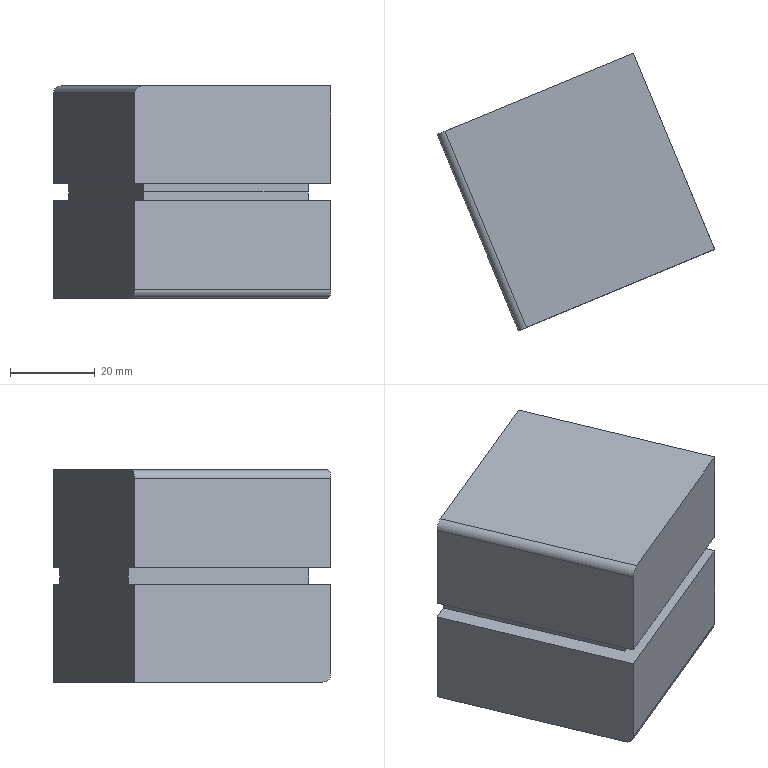Component | SolidWorks | Battery-2 | 1 solid | 17 faces | box 65.34 x 65.34 x 50 mm | volume 122620 mm3 | plane 15 | cylinder 2 | commonest cylinder face diameters 4 x2
build123d program:
from build123d import *

# Parameters (mm, degrees)
SKETCH1_W           = 50
SKETCH1_H           = 50
BOSS_EXTRUDE1_DEPTH = 50
SKETCH8_W           = 4
SKETCH8_H           = 4
FILLET1_R           = 2
FILLET4_R           = 2


with BuildPart() as part:
    # Sketch1 → Boss-Extrude1 (new body)
    with BuildSketch(Plane(origin=(0, 0, 0), x_dir=(1, 0, 0), z_dir=(0, 1, 0))):
        with Locations((0.8865, -4.255)):
            Rectangle(SKETCH1_W, SKETCH1_H)
    extrude(amount=BOSS_EXTRUDE1_DEPTH)

    # Cut-Sweep2: sweep along a path in Sketch2
    with BuildLine(Plane(origin=(25.887, 0, 0), x_dir=(0, 0, -1), z_dir=(1, 0, 0))) as cut_sweep2_path:
        Line((-4.255, 50), (-4.255, 0))
    # Sketch7 → Cut-Sweep2 (sweep, cut)
    with BuildSketch(Plane.XZ):
        Polygon((25.887, 4.255), (25.887, 6.255), (21.763, 6.255), (21.763, 2.255), (25.887, 2.255), align=None)
    sweep(path=cut_sweep2_path.line, mode=Mode.SUBTRACT)

    # Cut-Sweep3: sweep along a path in Sketch4
    with BuildLine(Plane.ZY.offset(24.113)) as cut_sweep3_path:
        Line((4.255, 50), (4.255, 0))
    # Sketch8 → Cut-Sweep3 (sweep, cut)
    with BuildSketch(Plane.XZ):
        with Locations((-22.117, 4.255)):
            Rectangle(SKETCH8_W, SKETCH8_H)
    sweep(path=cut_sweep3_path.line, mode=Mode.SUBTRACT)

    # Cut-Sweep4: sweep along a path in Sketch5
    with BuildLine(Plane.XZ) as cut_sweep4_path:
        Line((25.887, 4.255), (-24.113, 4.255))
    # Sketch10 → Cut-Sweep4 (sweep, cut)
    with BuildSketch(Plane(origin=(25.887, 0, 0), x_dir=(0, 0, -1), z_dir=(1, 0, 0))):
        Polygon((-2.255, 0), (-2.255, 4), (-4.255, 4), (-6.255, 4), (-6.255, 0), align=None)
    sweep(path=cut_sweep4_path.line, mode=Mode.SUBTRACT)

    # Fillet1
    fillet1_edges = [part.edges().sort_by_distance(p)[0] for p in [
        (-24.113, 25, 29.255),
    ]]
    fillet(fillet1_edges, radius=FILLET1_R)

    # Fillet4
    fillet4_edges = [part.edges().sort_by_distance(p)[0] for p in [
        (0.8865, 0, -20.745),
    ]]
    fillet(fillet4_edges, radius=FILLET4_R)


solid = part.part

# Placed as in the assembly
solid = solid.moved(Location((39.632, -16.373, 266.591), (0, 0, 22.523)))
STEP:
#1=COLOUR_RGB('',0.7922,0.8196,0.9333);
#2=FILL_AREA_STYLE_COLOUR('',#1);
#3=FILL_AREA_STYLE('',(#2));
#4=SURFACE_STYLE_FILL_AREA(#3);
#5=SURFACE_SIDE_STYLE('',(#4));
#6=SURFACE_STYLE_USAGE(.BOTH.,#5);
#7=PRESENTATION_STYLE_ASSIGNMENT((#6));
#8=CARTESIAN_POINT('',(0.7561,-0.9781,11.647));
#9=VERTEX_POINT('',#8);
#10=CARTESIAN_POINT('',(2.502,-0.2542,11.647));
#11=VERTEX_POINT('',#10);
#12=CARTESIAN_POINT('',(0.6834,-1.008,11.647));
#13=DIRECTION('',(0.9237,0.383,0.));
#14=VECTOR('',#13,39.37);
#15=LINE('',#12,#14);
#16=EDGE_CURVE('',#9,#11,#15,.T.);
#17=ORIENTED_EDGE('',*,*,#16,.F.);
#18=CARTESIAN_POINT('',(0.6834,-1.008,11.569));
#19=VERTEX_POINT('',#18);
#20=CARTESIAN_POINT('',(0.7561,-0.9781,11.569));
#21=DIRECTION('',(0.383,-0.9237,0.));
#22=DIRECTION('',(0.,0.,1.));
#23=AXIS2_PLACEMENT_3D('',#20,#21,#22);
#24=CIRCLE('',#23,0.07874);
#25=EDGE_CURVE('',#9,#19,#24,.T.);
#26=ORIENTED_EDGE('',*,*,#25,.T.);
#27=CARTESIAN_POINT('',(0.6834,-1.008,10.742));
#28=VERTEX_POINT('',#27);
#29=CARTESIAN_POINT('',(0.6834,-1.008,9.679));
#30=DIRECTION('',(-0.,-0.,1.));
#31=VECTOR('',#30,39.37);
#32=LINE('',#29,#31);
#33=EDGE_CURVE('',#28,#19,#32,.T.);
#34=ORIENTED_EDGE('',*,*,#33,.F.);
#35=CARTESIAN_POINT('',(2.502,-0.2542,10.742));
#36=VERTEX_POINT('',#35);
#37=CARTESIAN_POINT('',(2.502,-0.2542,10.742));
#38=DIRECTION('',(-0.9237,-0.383,-0.));
#39=VECTOR('',#38,39.37);
#40=LINE('',#37,#39);
#41=EDGE_CURVE('',#36,#28,#40,.T.);
#42=ORIENTED_EDGE('',*,*,#41,.F.);
#43=CARTESIAN_POINT('',(2.502,-0.2542,9.679));
#44=DIRECTION('',(0.,0.,-1.));
#45=VECTOR('',#44,39.37);
#46=LINE('',#43,#45);
#47=EDGE_CURVE('',#11,#36,#46,.T.);
#48=ORIENTED_EDGE('',*,*,#47,.F.);
#49=EDGE_LOOP('',(#17,#26,#34,#42,#48));
#50=FACE_OUTER_BOUND('',#49,.T.);
#51=CARTESIAN_POINT('',(1.56,-0.6446,10.496));
#52=DIRECTION('',(-0.383,0.9237,-0.));
#53=DIRECTION('',(-0.,-0.,1.));
#54=AXIS2_PLACEMENT_3D('',#51,#52,#53);
#55=PLANE('',#54);
#56=ADVANCED_FACE('',(#50),#55,.F.);
#57=CARTESIAN_POINT('',(2.291,-0.1709,10.584));
#58=VERTEX_POINT('',#57);
#59=CARTESIAN_POINT('',(2.291,-0.1709,10.663));
#60=VERTEX_POINT('',#59);
#61=CARTESIAN_POINT('',(2.291,-0.1709,10.742));
#62=DIRECTION('',(-0.,-0.,1.));
#63=VECTOR('',#62,39.37);
#64=LINE('',#61,#63);
#65=EDGE_CURVE('',#58,#60,#64,.T.);
#66=ORIENTED_EDGE('',*,*,#65,.F.);
#67=CARTESIAN_POINT('',(1.598,1.502,10.584));
#68=VERTEX_POINT('',#67);
#69=CARTESIAN_POINT('',(1.583,1.538,10.584));
#70=DIRECTION('',(0.383,-0.9237,-0.));
#71=VECTOR('',#70,39.37);
#72=LINE('',#69,#71);
#73=EDGE_CURVE('',#68,#58,#72,.T.);
#74=ORIENTED_EDGE('',*,*,#73,.F.);
#75=CARTESIAN_POINT('',(1.598,1.502,10.742));
#76=VERTEX_POINT('',#75);
#77=CARTESIAN_POINT('',(1.598,1.502,10.742));
#78=DIRECTION('',(0.,0.,-1.));
#79=VECTOR('',#78,39.37);
#80=LINE('',#77,#79);
#81=EDGE_CURVE('',#76,#68,#80,.T.);
#82=ORIENTED_EDGE('',*,*,#81,.F.);
#83=CARTESIAN_POINT('',(2.291,-0.1709,10.742));
#84=VERTEX_POINT('',#83);
#85=CARTESIAN_POINT('',(1.583,1.538,10.742));
#86=DIRECTION('',(0.383,-0.9237,-0.));
#87=VECTOR('',#86,39.37);
#88=LINE('',#85,#87);
#89=EDGE_CURVE('',#76,#84,#88,.T.);
#90=ORIENTED_EDGE('',*,*,#89,.T.);
#91=CARTESIAN_POINT('',(2.291,-0.1709,10.742));
#92=DIRECTION('',(-0.,-0.,1.));
#93=VECTOR('',#92,39.37);
#94=LINE('',#91,#93);
#95=EDGE_CURVE('',#60,#84,#94,.T.);
#96=ORIENTED_EDGE('',*,*,#95,.F.);
#97=EDGE_LOOP('',(#66,#74,#82,#90,#96));
#98=FACE_OUTER_BOUND('',#97,.T.);
#99=CARTESIAN_POINT('',(1.583,1.538,10.742));
#100=DIRECTION('',(-0.9237,-0.383,-0.));
#101=DIRECTION('',(-0.,-0.,1.));
#102=AXIS2_PLACEMENT_3D('',#99,#100,#101);
#103=PLANE('',#102);
#104=ADVANCED_FACE('',(#98),#103,.F.);
#105=CARTESIAN_POINT('',(0.7684,-0.8025,10.663));
#106=VERTEX_POINT('',#105);
#107=CARTESIAN_POINT('',(0.7684,-0.8025,10.584));
#108=VERTEX_POINT('',#107);
#109=CARTESIAN_POINT('',(0.7684,-0.8025,10.742));
#110=DIRECTION('',(0.,0.,-1.));
#111=VECTOR('',#110,39.37);
#112=LINE('',#109,#111);
#113=EDGE_CURVE('',#106,#108,#112,.T.);
#114=ORIENTED_EDGE('',*,*,#113,.F.);
#115=CARTESIAN_POINT('',(0.7684,-0.8025,10.742));
#116=VERTEX_POINT('',#115);
#117=CARTESIAN_POINT('',(0.7684,-0.8025,10.742));
#118=DIRECTION('',(0.,0.,-1.));
#119=VECTOR('',#118,39.37);
#120=LINE('',#117,#119);
#121=EDGE_CURVE('',#116,#106,#120,.T.);
#122=ORIENTED_EDGE('',*,*,#121,.F.);
#123=CARTESIAN_POINT('',(0.07469,0.8704,10.742));
#124=VERTEX_POINT('',#123);
#125=CARTESIAN_POINT('',(0.05961,0.9067,10.742));
#126=DIRECTION('',(0.383,-0.9237,-0.));
#127=VECTOR('',#126,39.37);
#128=LINE('',#125,#127);
#129=EDGE_CURVE('',#124,#116,#128,.T.);
#130=ORIENTED_EDGE('',*,*,#129,.F.);
#131=CARTESIAN_POINT('',(0.07469,0.8704,10.584));
#132=VERTEX_POINT('',#131);
#133=CARTESIAN_POINT('',(0.07469,0.8704,10.742));
#134=DIRECTION('',(-0.,-0.,1.));
#135=VECTOR('',#134,39.37);
#136=LINE('',#133,#135);
#137=EDGE_CURVE('',#132,#124,#136,.T.);
#138=ORIENTED_EDGE('',*,*,#137,.F.);
#139=CARTESIAN_POINT('',(0.05961,0.9067,10.584));
#140=DIRECTION('',(0.383,-0.9237,-0.));
#141=VECTOR('',#140,39.37);
#142=LINE('',#139,#141);
#143=EDGE_CURVE('',#132,#108,#142,.T.);
#144=ORIENTED_EDGE('',*,*,#143,.T.);
#145=EDGE_LOOP('',(#114,#122,#130,#138,#144));
#146=FACE_OUTER_BOUND('',#145,.T.);
#147=CARTESIAN_POINT('',(0.05961,0.9067,10.742));
#148=DIRECTION('',(0.9237,0.383,0.));
#149=DIRECTION('',(0.,0.,-1.));
#150=AXIS2_PLACEMENT_3D('',#147,#148,#149);
#151=PLANE('',#150);
#152=ADVANCED_FACE('',(#146),#151,.F.);
#153=ORIENTED_EDGE('',*,*,#33,.T.);
#154=CARTESIAN_POINT('',(-0.07064,0.8101,11.569));
#155=VERTEX_POINT('',#154);
#156=CARTESIAN_POINT('',(-0.07064,0.8101,11.569));
#157=DIRECTION('',(-0.383,0.9237,-0.));
#158=VECTOR('',#157,39.37);
#159=LINE('',#156,#158);
#160=EDGE_CURVE('',#19,#155,#159,.T.);
#161=ORIENTED_EDGE('',*,*,#160,.T.);
#162=CARTESIAN_POINT('',(-0.07064,0.8101,10.742));
#163=VERTEX_POINT('',#162);
#164=CARTESIAN_POINT('',(-0.07064,0.8101,9.679));
#165=DIRECTION('',(-0.,-0.,1.));
#166=VECTOR('',#165,39.37);
#167=LINE('',#164,#166);
#168=EDGE_CURVE('',#163,#155,#167,.T.);
#169=ORIENTED_EDGE('',*,*,#168,.F.);
#170=CARTESIAN_POINT('',(-0.07064,0.8101,10.742));
#171=DIRECTION('',(0.383,-0.9237,-0.));
#172=VECTOR('',#171,39.37);
#173=LINE('',#170,#172);
#174=EDGE_CURVE('',#163,#28,#173,.T.);
#175=ORIENTED_EDGE('',*,*,#174,.T.);
#176=EDGE_LOOP('',(#153,#161,#169,#175));
#177=FACE_OUTER_BOUND('',#176,.T.);
#178=CARTESIAN_POINT('',(-0.07064,0.8101,9.679));
#179=DIRECTION('',(0.9237,0.383,0.));
#180=DIRECTION('',(0.,0.,-1.));
#181=AXIS2_PLACEMENT_3D('',#178,#179,#180);
#182=PLANE('',#181);
#183=ADVANCED_FACE('',(#177),#182,.F.);
#184=CARTESIAN_POINT('',(2.502,-0.2542,10.584));
#185=VERTEX_POINT('',#184);
#186=CARTESIAN_POINT('',(2.502,-0.2542,9.758));
#187=VERTEX_POINT('',#186);
#188=CARTESIAN_POINT('',(2.502,-0.2542,9.679));
#189=DIRECTION('',(0.,0.,-1.));
#190=VECTOR('',#189,39.37);
#191=LINE('',#188,#190);
#192=EDGE_CURVE('',#185,#187,#191,.T.);
#193=ORIENTED_EDGE('',*,*,#192,.T.);
#194=CARTESIAN_POINT('',(2.472,-0.1815,9.679));
#195=VERTEX_POINT('',#194);
#196=CARTESIAN_POINT('',(2.472,-0.1815,9.758));
#197=DIRECTION('',(0.9237,0.383,0.));
#198=DIRECTION('',(0.,0.,1.));
#199=AXIS2_PLACEMENT_3D('',#196,#197,#198);
#200=CIRCLE('',#199,0.07874);
#201=EDGE_CURVE('',#187,#195,#200,.T.);
#202=ORIENTED_EDGE('',*,*,#201,.T.);
#203=CARTESIAN_POINT('',(1.748,1.564,9.679));
#204=VERTEX_POINT('',#203);
#205=CARTESIAN_POINT('',(1.748,1.564,9.679));
#206=DIRECTION('',(0.383,-0.9237,0.));
#207=VECTOR('',#206,39.37);
#208=LINE('',#205,#207);
#209=EDGE_CURVE('',#204,#195,#208,.T.);
#210=ORIENTED_EDGE('',*,*,#209,.F.);
#211=CARTESIAN_POINT('',(1.748,1.564,10.584));
#212=VERTEX_POINT('',#211);
#213=CARTESIAN_POINT('',(1.748,1.564,9.679));
#214=DIRECTION('',(0.,0.,-1.));
#215=VECTOR('',#214,39.37);
#216=LINE('',#213,#215);
#217=EDGE_CURVE('',#212,#204,#216,.T.);
#218=ORIENTED_EDGE('',*,*,#217,.F.);
#219=CARTESIAN_POINT('',(1.733,1.601,10.584));
#220=DIRECTION('',(0.383,-0.9237,-0.));
#221=VECTOR('',#220,39.37);
#222=LINE('',#219,#221);
#223=EDGE_CURVE('',#212,#185,#222,.T.);
#224=ORIENTED_EDGE('',*,*,#223,.T.);
#225=EDGE_LOOP('',(#193,#202,#210,#218,#224));
#226=FACE_OUTER_BOUND('',#225,.T.);
#227=CARTESIAN_POINT('',(1.748,1.564,9.679));
#228=DIRECTION('',(-0.9237,-0.383,-0.));
#229=DIRECTION('',(-0.,-0.,1.));
#230=AXIS2_PLACEMENT_3D('',#227,#228,#229);
#231=PLANE('',#230);
#232=ADVANCED_FACE('',(#226),#231,.F.);
#233=CARTESIAN_POINT('',(-0.07064,0.8101,9.679));
#234=VERTEX_POINT('',#233);
#235=CARTESIAN_POINT('',(0.6532,-0.9355,9.679));
#236=VERTEX_POINT('',#235);
#237=CARTESIAN_POINT('',(-0.07064,0.8101,9.679));
#238=DIRECTION('',(0.383,-0.9237,0.));
#239=VECTOR('',#238,39.37);
#240=LINE('',#237,#239);
#241=EDGE_CURVE('',#234,#236,#240,.T.);
#242=ORIENTED_EDGE('',*,*,#241,.T.);
#243=CARTESIAN_POINT('',(0.6834,-1.008,9.758));
#244=VERTEX_POINT('',#243);
#245=CARTESIAN_POINT('',(0.6532,-0.9355,9.758));
#246=DIRECTION('',(-0.9237,-0.383,-0.));
#247=DIRECTION('',(0.,0.,-1.));
#248=AXIS2_PLACEMENT_3D('',#245,#246,#247);
#249=CIRCLE('',#248,0.07874);
#250=EDGE_CURVE('',#236,#244,#249,.T.);
#251=ORIENTED_EDGE('',*,*,#250,.T.);
#252=CARTESIAN_POINT('',(0.6834,-1.008,10.584));
#253=VERTEX_POINT('',#252);
#254=CARTESIAN_POINT('',(0.6834,-1.008,9.679));
#255=DIRECTION('',(-0.,-0.,1.));
#256=VECTOR('',#255,39.37);
#257=LINE('',#254,#256);
#258=EDGE_CURVE('',#244,#253,#257,.T.);
#259=ORIENTED_EDGE('',*,*,#258,.T.);
#260=CARTESIAN_POINT('',(-0.07064,0.8101,10.584));
#261=VERTEX_POINT('',#260);
#262=CARTESIAN_POINT('',(-0.07064,0.8101,10.584));
#263=DIRECTION('',(-0.383,0.9237,0.));
#264=VECTOR('',#263,39.37);
#265=LINE('',#262,#264);
#266=EDGE_CURVE('',#253,#261,#265,.T.);
#267=ORIENTED_EDGE('',*,*,#266,.T.);
#268=CARTESIAN_POINT('',(-0.07064,0.8101,9.679));
#269=DIRECTION('',(-0.,-0.,1.));
#270=VECTOR('',#269,39.37);
#271=LINE('',#268,#270);
#272=EDGE_CURVE('',#234,#261,#271,.T.);
#273=ORIENTED_EDGE('',*,*,#272,.F.);
#274=EDGE_LOOP('',(#242,#251,#259,#267,#273));
#275=FACE_OUTER_BOUND('',#274,.T.);
#276=CARTESIAN_POINT('',(-0.07064,0.8101,9.679));
#277=DIRECTION('',(0.9237,0.383,0.));
#278=DIRECTION('',(0.,0.,-1.));
#279=AXIS2_PLACEMENT_3D('',#276,#277,#278);
#280=PLANE('',#279);
#281=ADVANCED_FACE('',(#275),#280,.F.);
#282=CARTESIAN_POINT('',(0.002094,0.8403,11.647));
#283=VERTEX_POINT('',#282);
#284=CARTESIAN_POINT('',(1.748,1.564,11.647));
#285=VERTEX_POINT('',#284);
#286=CARTESIAN_POINT('',(-0.07064,0.8101,11.647));
#287=DIRECTION('',(0.9237,0.383,0.));
#288=VECTOR('',#287,39.37);
#289=LINE('',#286,#288);
#290=EDGE_CURVE('',#283,#285,#289,.T.);
#291=ORIENTED_EDGE('',*,*,#290,.F.);
#292=CARTESIAN_POINT('',(0.002094,0.8403,11.647));
#293=DIRECTION('',(0.383,-0.9237,0.));
#294=VECTOR('',#293,39.37);
#295=LINE('',#292,#294);
#296=EDGE_CURVE('',#283,#9,#295,.T.);
#297=ORIENTED_EDGE('',*,*,#296,.T.);
#298=ORIENTED_EDGE('',*,*,#16,.T.);
#299=CARTESIAN_POINT('',(1.748,1.564,11.647));
#300=DIRECTION('',(0.383,-0.9237,0.));
#301=VECTOR('',#300,39.37);
#302=LINE('',#299,#301);
#303=EDGE_CURVE('',#285,#11,#302,.T.);
#304=ORIENTED_EDGE('',*,*,#303,.F.);
#305=EDGE_LOOP('',(#291,#297,#298,#304));
#306=FACE_OUTER_BOUND('',#305,.T.);
#307=CARTESIAN_POINT('',(-0.07064,0.8101,11.647));
#308=DIRECTION('',(0.,0.,-1.));
#309=DIRECTION('',(-0.9237,-0.383,-0.));
#310=AXIS2_PLACEMENT_3D('',#307,#308,#309);
#311=PLANE('',#310);
#312=ADVANCED_FACE('',(#306),#311,.F.);
#313=ORIENTED_EDGE('',*,*,#47,.T.);
#314=CARTESIAN_POINT('',(1.748,1.564,10.742));
#315=VERTEX_POINT('',#314);
#316=CARTESIAN_POINT('',(1.733,1.601,10.742));
#317=DIRECTION('',(0.383,-0.9237,-0.));
#318=VECTOR('',#317,39.37);
#319=LINE('',#316,#318);
#320=EDGE_CURVE('',#315,#36,#319,.T.);
#321=ORIENTED_EDGE('',*,*,#320,.F.);
#322=CARTESIAN_POINT('',(1.748,1.564,9.679));
#323=DIRECTION('',(0.,0.,-1.));
#324=VECTOR('',#323,39.37);
#325=LINE('',#322,#324);
#326=EDGE_CURVE('',#285,#315,#325,.T.);
#327=ORIENTED_EDGE('',*,*,#326,.F.);
#328=ORIENTED_EDGE('',*,*,#303,.T.);
#329=EDGE_LOOP('',(#313,#321,#327,#328));
#330=FACE_OUTER_BOUND('',#329,.T.);
#331=CARTESIAN_POINT('',(1.748,1.564,9.679));
#332=DIRECTION('',(-0.9237,-0.383,-0.));
#333=DIRECTION('',(-0.,-0.,1.));
#334=AXIS2_PLACEMENT_3D('',#331,#332,#333);
#335=PLANE('',#334);
#336=ADVANCED_FACE('',(#330),#335,.F.);
#337=ORIENTED_EDGE('',*,*,#209,.T.);
#338=CARTESIAN_POINT('',(0.6532,-0.9355,9.679));
#339=DIRECTION('',(-0.9237,-0.383,-0.));
#340=VECTOR('',#339,39.37);
#341=LINE('',#338,#340);
#342=EDGE_CURVE('',#195,#236,#341,.T.);
#343=ORIENTED_EDGE('',*,*,#342,.T.);
#344=ORIENTED_EDGE('',*,*,#241,.F.);
#345=CARTESIAN_POINT('',(-0.07064,0.8101,9.679));
#346=DIRECTION('',(-0.9237,-0.383,-0.));
#347=VECTOR('',#346,39.37);
#348=LINE('',#345,#347);
#349=EDGE_CURVE('',#204,#234,#348,.T.);
#350=ORIENTED_EDGE('',*,*,#349,.F.);
#351=EDGE_LOOP('',(#337,#343,#344,#350));
#352=FACE_OUTER_BOUND('',#351,.T.);
#353=CARTESIAN_POINT('',(-0.07064,0.8101,9.679));
#354=DIRECTION('',(-0.,-0.,1.));
#355=DIRECTION('',(0.9237,0.383,0.));
#356=AXIS2_PLACEMENT_3D('',#353,#354,#355);
#357=PLANE('',#356);
#358=ADVANCED_FACE('',(#352),#357,.F.);
#359=ORIENTED_EDGE('',*,*,#168,.T.);
#360=CARTESIAN_POINT('',(0.002094,0.8403,11.569));
#361=DIRECTION('',(-0.383,0.9237,-0.));
#362=DIRECTION('',(-0.,0.,1.));
#363=AXIS2_PLACEMENT_3D('',#360,#361,#362);
#364=CIRCLE('',#363,0.07874);
#365=EDGE_CURVE('',#155,#283,#364,.T.);
#366=ORIENTED_EDGE('',*,*,#365,.T.);
#367=ORIENTED_EDGE('',*,*,#290,.T.);
#368=ORIENTED_EDGE('',*,*,#326,.T.);
#369=CARTESIAN_POINT('',(1.748,1.564,10.742));
#370=DIRECTION('',(-0.9237,-0.383,-0.));
#371=VECTOR('',#370,39.37);
#372=LINE('',#369,#371);
#373=EDGE_CURVE('',#315,#76,#372,.T.);
#374=ORIENTED_EDGE('',*,*,#373,.T.);
#375=ORIENTED_EDGE('',*,*,#81,.T.);
#376=CARTESIAN_POINT('',(1.598,1.502,10.584));
#377=DIRECTION('',(0.9237,0.383,0.));
#378=VECTOR('',#377,39.37);
#379=LINE('',#376,#378);
#380=EDGE_CURVE('',#68,#212,#379,.T.);
#381=ORIENTED_EDGE('',*,*,#380,.T.);
#382=ORIENTED_EDGE('',*,*,#217,.T.);
#383=ORIENTED_EDGE('',*,*,#349,.T.);
#384=ORIENTED_EDGE('',*,*,#272,.T.);
#385=CARTESIAN_POINT('',(-0.07078,0.8101,10.584));
#386=DIRECTION('',(0.9237,0.383,0.));
#387=VECTOR('',#386,39.37);
#388=LINE('',#385,#387);
#389=EDGE_CURVE('',#261,#132,#388,.T.);
#390=ORIENTED_EDGE('',*,*,#389,.T.);
#391=ORIENTED_EDGE('',*,*,#137,.T.);
#392=CARTESIAN_POINT('',(0.07469,0.8704,10.742));
#393=DIRECTION('',(-0.9237,-0.383,-0.));
#394=VECTOR('',#393,39.37);
#395=LINE('',#392,#394);
#396=EDGE_CURVE('',#124,#163,#395,.T.);
#397=ORIENTED_EDGE('',*,*,#396,.T.);
#398=EDGE_LOOP('',(#359,#366,#367,#368,#374,#375,#381,#382,#383,#384,#390,#391,#397));
#399=FACE_OUTER_BOUND('',#398,.T.);
#400=CARTESIAN_POINT('',(0.8063,1.174,10.496));
#401=DIRECTION('',(-0.383,0.9237,-0.));
#402=DIRECTION('',(-0.,-0.,1.));
#403=AXIS2_PLACEMENT_3D('',#400,#401,#402);
#404=PLANE('',#403);
#405=ADVANCED_FACE('',(#399),#404,.T.);
#406=ORIENTED_EDGE('',*,*,#258,.F.);
#407=CARTESIAN_POINT('',(1.56,-0.6446,9.758));
#408=DIRECTION('',(0.9237,0.383,0.));
#409=VECTOR('',#408,39.37);
#410=LINE('',#407,#409);
#411=EDGE_CURVE('',#244,#187,#410,.T.);
#412=ORIENTED_EDGE('',*,*,#411,.T.);
#413=ORIENTED_EDGE('',*,*,#192,.F.);
#414=CARTESIAN_POINT('',(2.352,-0.3164,10.584));
#415=DIRECTION('',(0.9237,0.383,0.));
#416=VECTOR('',#415,39.37);
#417=LINE('',#414,#416);
#418=EDGE_CURVE('',#253,#185,#417,.T.);
#419=ORIENTED_EDGE('',*,*,#418,.F.);
#420=EDGE_LOOP('',(#406,#412,#413,#419));
#421=FACE_OUTER_BOUND('',#420,.T.);
#422=CARTESIAN_POINT('',(1.56,-0.6446,10.496));
#423=DIRECTION('',(-0.383,0.9237,-0.));
#424=DIRECTION('',(-0.,-0.,1.));
#425=AXIS2_PLACEMENT_3D('',#422,#423,#424);
#426=PLANE('',#425);
#427=ADVANCED_FACE('',(#421),#426,.F.);
#428=ORIENTED_EDGE('',*,*,#418,.T.);
#429=ORIENTED_EDGE('',*,*,#223,.F.);
#430=ORIENTED_EDGE('',*,*,#380,.F.);
#431=ORIENTED_EDGE('',*,*,#73,.T.);
#432=CARTESIAN_POINT('',(2.441,-0.1087,10.584));
#433=DIRECTION('',(-0.9237,-0.383,-0.));
#434=VECTOR('',#433,39.37);
#435=LINE('',#432,#434);
#436=EDGE_CURVE('',#58,#108,#435,.T.);
#437=ORIENTED_EDGE('',*,*,#436,.T.);
#438=ORIENTED_EDGE('',*,*,#143,.F.);
#439=ORIENTED_EDGE('',*,*,#389,.F.);
#440=ORIENTED_EDGE('',*,*,#266,.F.);
#441=EDGE_LOOP('',(#428,#429,#430,#431,#437,#438,#439,#440));
#442=FACE_OUTER_BOUND('',#441,.T.);
#443=CARTESIAN_POINT('',(1.583,1.538,10.584));
#444=DIRECTION('',(0.,0.,-1.));
#445=DIRECTION('',(-0.383,0.9237,0.));
#446=AXIS2_PLACEMENT_3D('',#443,#444,#445);
#447=PLANE('',#446);
#448=ADVANCED_FACE('',(#442),#447,.F.);
#449=ORIENTED_EDGE('',*,*,#320,.T.);
#450=ORIENTED_EDGE('',*,*,#41,.T.);
#451=ORIENTED_EDGE('',*,*,#174,.F.);
#452=ORIENTED_EDGE('',*,*,#396,.F.);
#453=ORIENTED_EDGE('',*,*,#129,.T.);
#454=CARTESIAN_POINT('',(2.441,-0.1087,10.742));
#455=DIRECTION('',(-0.9237,-0.383,-0.));
#456=VECTOR('',#455,39.37);
#457=LINE('',#454,#456);
#458=EDGE_CURVE('',#84,#116,#457,.T.);
#459=ORIENTED_EDGE('',*,*,#458,.F.);
#460=ORIENTED_EDGE('',*,*,#89,.F.);
#461=ORIENTED_EDGE('',*,*,#373,.F.);
#462=EDGE_LOOP('',(#449,#450,#451,#452,#453,#459,#460,#461));
#463=FACE_OUTER_BOUND('',#462,.T.);
#464=CARTESIAN_POINT('',(1.733,1.601,10.742));
#465=DIRECTION('',(-0.,-0.,1.));
#466=DIRECTION('',(0.383,-0.9237,-0.));
#467=AXIS2_PLACEMENT_3D('',#464,#465,#466);
#468=PLANE('',#467);
#469=ADVANCED_FACE('',(#463),#468,.F.);
#470=ORIENTED_EDGE('',*,*,#65,.T.);
#471=CARTESIAN_POINT('',(2.441,-0.1087,10.663));
#472=DIRECTION('',(-0.9237,-0.383,-0.));
#473=VECTOR('',#472,39.37);
#474=LINE('',#471,#473);
#475=EDGE_CURVE('',#60,#106,#474,.T.);
#476=ORIENTED_EDGE('',*,*,#475,.T.);
#477=ORIENTED_EDGE('',*,*,#113,.T.);
#478=ORIENTED_EDGE('',*,*,#436,.F.);
#479=EDGE_LOOP('',(#470,#476,#477,#478));
#480=FACE_OUTER_BOUND('',#479,.T.);
#481=CARTESIAN_POINT('',(2.441,-0.1087,10.584));
#482=DIRECTION('',(0.383,-0.9237,0.));
#483=DIRECTION('',(0.,0.,-1.));
#484=AXIS2_PLACEMENT_3D('',#481,#482,#483);
#485=PLANE('',#484);
#486=ADVANCED_FACE('',(#480),#485,.T.);
#487=ORIENTED_EDGE('',*,*,#95,.T.);
#488=ORIENTED_EDGE('',*,*,#458,.T.);
#489=ORIENTED_EDGE('',*,*,#121,.T.);
#490=ORIENTED_EDGE('',*,*,#475,.F.);
#491=EDGE_LOOP('',(#487,#488,#489,#490));
#492=FACE_OUTER_BOUND('',#491,.T.);
#493=CARTESIAN_POINT('',(2.441,-0.1087,10.663));
#494=DIRECTION('',(0.383,-0.9237,0.));
#495=DIRECTION('',(0.,0.,-1.));
#496=AXIS2_PLACEMENT_3D('',#493,#494,#495);
#497=PLANE('',#496);
#498=ADVANCED_FACE('',(#492),#497,.T.);
#499=ORIENTED_EDGE('',*,*,#365,.F.);
#500=ORIENTED_EDGE('',*,*,#160,.F.);
#501=ORIENTED_EDGE('',*,*,#25,.F.);
#502=ORIENTED_EDGE('',*,*,#296,.F.);
#503=EDGE_LOOP('',(#499,#500,#501,#502));
#504=FACE_OUTER_BOUND('',#503,.T.);
#505=CARTESIAN_POINT('',(0.002094,0.8403,11.569));
#506=DIRECTION('',(0.383,-0.9237,0.));
#507=DIRECTION('',(0.,0.,-1.));
#508=AXIS2_PLACEMENT_3D('',#505,#506,#507);
#509=CYLINDRICAL_SURFACE('',#508,0.07874);
#510=ADVANCED_FACE('',(#504),#509,.T.);
#511=ORIENTED_EDGE('',*,*,#201,.F.);
#512=ORIENTED_EDGE('',*,*,#411,.F.);
#513=ORIENTED_EDGE('',*,*,#250,.F.);
#514=ORIENTED_EDGE('',*,*,#342,.F.);
#515=EDGE_LOOP('',(#511,#512,#513,#514));
#516=FACE_OUTER_BOUND('',#515,.T.);
#517=CARTESIAN_POINT('',(0.6532,-0.9355,9.758));
#518=DIRECTION('',(-0.9237,-0.383,-0.));
#519=DIRECTION('',(0.,0.,1.));
#520=AXIS2_PLACEMENT_3D('',#517,#518,#519);
#521=CYLINDRICAL_SURFACE('',#520,0.07874);
#522=ADVANCED_FACE('',(#516),#521,.T.);
#523=CLOSED_SHELL('',(#56,#104,#152,#183,#232,#281,#312,#336,#358,#405,#427,#448,#469,#486,#498,#510,#522));
#524=MANIFOLD_SOLID_BREP('',#523);
#525=STYLED_ITEM('',(#7),#524);
#526=(LENGTH_UNIT()NAMED_UNIT(*)SI_UNIT($,.METRE.));
#527=LENGTH_MEASURE_WITH_UNIT(LENGTH_MEASURE(0.0254),#526);
#528=DIMENSIONAL_EXPONENTS(1.,0.,0.,0.,0.,0.,0.);
#529=(CONVERSION_BASED_UNIT('',#527)LENGTH_UNIT()NAMED_UNIT(#528));
#530=UNCERTAINTY_MEASURE_WITH_UNIT(LENGTH_MEASURE(0.00001),#529,'','');
#531=(NAMED_UNIT(*)PLANE_ANGLE_UNIT()SI_UNIT($,.RADIAN.));
#532=(NAMED_UNIT(*)SI_UNIT($,.STERADIAN.)SOLID_ANGLE_UNIT());
#533=(GEOMETRIC_REPRESENTATION_CONTEXT(3)GLOBAL_UNCERTAINTY_ASSIGNED_CONTEXT((#530))GLOBAL_UNIT_ASSIGNED_CONTEXT((#529,#531,#532))REPRESENTATION_CONTEXT('',''));
#534=MECHANICAL_DESIGN_GEOMETRIC_PRESENTATION_REPRESENTATION('',(#525),#533);
#535=CARTESIAN_POINT('',(0.,0.,0.));
#536=DIRECTION('',(0.,0.,1.));
#537=DIRECTION('',(1.,0.,0.));
#538=AXIS2_PLACEMENT_3D('',#535,#536,#537);
#539=(LENGTH_UNIT()NAMED_UNIT(*)SI_UNIT($,.METRE.));
#540=LENGTH_MEASURE_WITH_UNIT(LENGTH_MEASURE(0.0254),#539);
#541=DIMENSIONAL_EXPONENTS(1.,0.,0.,0.,0.,0.,0.);
#542=(CONVERSION_BASED_UNIT('',#540)LENGTH_UNIT()NAMED_UNIT(#541));
#543=UNCERTAINTY_MEASURE_WITH_UNIT(LENGTH_MEASURE(0.00001),#542,'','');
#544=(NAMED_UNIT(*)PLANE_ANGLE_UNIT()SI_UNIT($,.RADIAN.));
#545=(NAMED_UNIT(*)SI_UNIT($,.STERADIAN.)SOLID_ANGLE_UNIT());
#546=(GEOMETRIC_REPRESENTATION_CONTEXT(3)GLOBAL_UNCERTAINTY_ASSIGNED_CONTEXT((#543))GLOBAL_UNIT_ASSIGNED_CONTEXT((#542,#544,#545))REPRESENTATION_CONTEXT('',''));
#547=ADVANCED_BREP_SHAPE_REPRESENTATION('',(#524,#538),#546);
#548=PRESENTATION_LAYER_ASSIGNMENT('','',(#525));